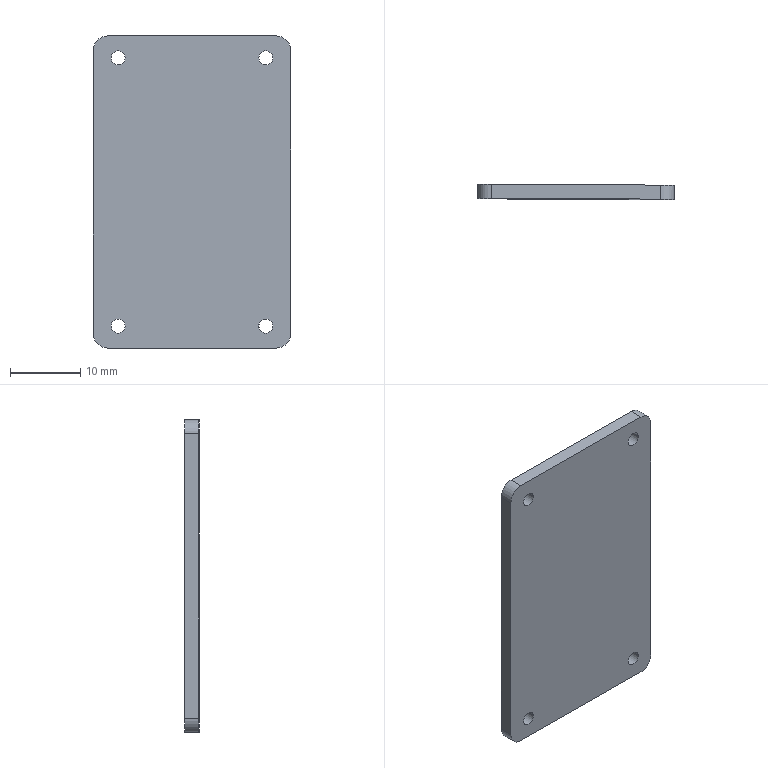Component | SolidWorks | LowerBaffle-1 | 1 solid | 23 faces | box 28.12 x 2.12 x 44.53 mm | volume 2302 mm3 | cylinder 12 | plane 11 | commonest cylinder face diameters 2 x8 4 x4
build123d program:
from build123d import *

# Parameters (mm, degrees)
BOSS_EXTRUDE1_DEPTH = 2
FILLET1_R           = 2
SKETCH2_R           = 1
CUT_EXTRUDE1_DEPTH  = 10
SKETCH3_W           = 14.313
SKETCH3_H           = 23.58
CUT_EXTRUDE2_DEPTH  = 0.5


with BuildPart() as part:
    # Sketch1 → Boss-Extrude1 (new body)
    with BuildSketch(Plane.XY):
        Polygon((102.385, 21.878), (74.276, 21.878), (74.276, -0.3844), (74.276, -22.646), (102.385, -22.646), align=None)
    extrude(amount=BOSS_EXTRUDE1_DEPTH)

    # Fillet1
    fillet1_edges = [part.edges().sort_by_distance(p)[0] for p in [
        (102.385, -22.646, 1),
        (74.276, -22.646, 1),
        (74.276, 21.878, 1),
        (102.385, 21.878, 1),
    ]]
    fillet(fillet1_edges, radius=FILLET1_R)

    # Sketch2 → Cut-Extrude1 (cut)
    with BuildSketch(Plane.XY.offset(2)):
        with Locations((98.864, 18.749)):
            Circle(SKETCH2_R)
        with Locations((77.792, 18.749)):
            Circle(SKETCH2_R)
        with Locations(Location((77.792, -19.518, 0), (0, 0, 180))):
            Circle(SKETCH2_R)
        with Locations(Location((98.864, -19.518, 0), (0, 0, 180))):
            Circle(SKETCH2_R)
    extrude(amount=-CUT_EXTRUDE1_DEPTH, mode=Mode.SUBTRACT)

    # Sketch3 → Cut-Extrude2 (cut)
    with BuildSketch(Plane.XY.offset(2)):
        with Locations((89.245, -0.1111)):
            Rectangle(SKETCH3_W, SKETCH3_H)
    extrude(amount=-CUT_EXTRUDE2_DEPTH, mode=Mode.SUBTRACT)


solid = part.part

# Placed as in the assembly
solid = solid.moved(Location((64.806, 26.824, -0.2506), (-90, 0.2356, 0.008241)))
STEP:
#1=COLOUR_RGB('',0.7922,0.8196,0.9333);
#2=FILL_AREA_STYLE_COLOUR('',#1);
#3=FILL_AREA_STYLE('',(#2));
#4=SURFACE_STYLE_FILL_AREA(#3);
#5=SURFACE_SIDE_STYLE('',(#4));
#6=SURFACE_STYLE_USAGE(.BOTH.,#5);
#7=PRESENTATION_STYLE_ASSIGNMENT((#6));
#8=CARTESIAN_POINT('',(6.483,1.04,0.758));
#9=VERTEX_POINT('',#8);
#10=CARTESIAN_POINT('',(6.404,1.04,0.758));
#11=VERTEX_POINT('',#10);
#12=CARTESIAN_POINT('',(6.444,1.04,0.758));
#13=DIRECTION('',(-0.004111,-1.,0.));
#14=DIRECTION('',(-1.,0.004111,0.0001438));
#15=AXIS2_PLACEMENT_3D('',#12,#13,#14);
#16=CIRCLE('',#15,0.03937);
#17=EDGE_CURVE('',#9,#11,#16,.T.);
#18=ORIENTED_EDGE('',*,*,#17,.T.);
#19=CARTESIAN_POINT('',(6.405,1.119,0.758));
#20=VERTEX_POINT('',#19);
#21=CARTESIAN_POINT('',(6.403,0.7253,0.758));
#22=DIRECTION('',(0.004111,1.,0.));
#23=VECTOR('',#22,39.37);
#24=LINE('',#21,#23);
#25=EDGE_CURVE('',#11,#20,#24,.T.);
#26=ORIENTED_EDGE('',*,*,#25,.T.);
#27=CARTESIAN_POINT('',(6.483,1.119,0.758));
#28=VERTEX_POINT('',#27);
#29=CARTESIAN_POINT('',(6.444,1.119,0.758));
#30=DIRECTION('',(0.004111,1.,0.));
#31=DIRECTION('',(-1.,0.004111,0.0001438));
#32=AXIS2_PLACEMENT_3D('',#29,#30,#31);
#33=CIRCLE('',#32,0.03937);
#34=EDGE_CURVE('',#20,#28,#33,.T.);
#35=ORIENTED_EDGE('',*,*,#34,.T.);
#36=CARTESIAN_POINT('',(6.482,0.7249,0.758));
#37=DIRECTION('',(0.004111,1.,0.));
#38=VECTOR('',#37,39.37);
#39=LINE('',#36,#38);
#40=EDGE_CURVE('',#9,#28,#39,.T.);
#41=ORIENTED_EDGE('',*,*,#40,.F.);
#42=EDGE_LOOP('',(#18,#26,#35,#41));
#43=FACE_OUTER_BOUND('',#42,.T.);
#44=CARTESIAN_POINT('',(6.442,0.7251,0.758));
#45=DIRECTION('',(0.004111,1.,0.));
#46=DIRECTION('',(1.,-0.004111,-0.0001438));
#47=AXIS2_PLACEMENT_3D('',#44,#45,#46);
#48=CYLINDRICAL_SURFACE('',#47,0.03937);
#49=ADVANCED_FACE('',(#43),#48,.F.);
#50=CARTESIAN_POINT('',(5.654,1.043,0.7581));
#51=VERTEX_POINT('',#50);
#52=CARTESIAN_POINT('',(5.575,1.044,0.7581));
#53=VERTEX_POINT('',#52);
#54=CARTESIAN_POINT('',(5.614,1.043,0.7581));
#55=DIRECTION('',(-0.004111,-1.,0.));
#56=DIRECTION('',(-1.,0.004111,0.0001438));
#57=AXIS2_PLACEMENT_3D('',#54,#55,#56);
#58=CIRCLE('',#57,0.03937);
#59=EDGE_CURVE('',#51,#53,#58,.T.);
#60=ORIENTED_EDGE('',*,*,#59,.T.);
#61=CARTESIAN_POINT('',(5.575,1.122,0.7581));
#62=VERTEX_POINT('',#61);
#63=CARTESIAN_POINT('',(5.573,0.7287,0.7581));
#64=DIRECTION('',(0.004111,1.,0.));
#65=VECTOR('',#64,39.37);
#66=LINE('',#63,#65);
#67=EDGE_CURVE('',#53,#62,#66,.T.);
#68=ORIENTED_EDGE('',*,*,#67,.T.);
#69=CARTESIAN_POINT('',(5.654,1.122,0.7581));
#70=VERTEX_POINT('',#69);
#71=CARTESIAN_POINT('',(5.614,1.122,0.7581));
#72=DIRECTION('',(0.004111,1.,0.));
#73=DIRECTION('',(-1.,0.004111,0.0001438));
#74=AXIS2_PLACEMENT_3D('',#71,#72,#73);
#75=CIRCLE('',#74,0.03937);
#76=EDGE_CURVE('',#62,#70,#75,.T.);
#77=ORIENTED_EDGE('',*,*,#76,.T.);
#78=CARTESIAN_POINT('',(5.652,0.7284,0.7581));
#79=DIRECTION('',(0.004111,1.,0.));
#80=VECTOR('',#79,39.37);
#81=LINE('',#78,#80);
#82=EDGE_CURVE('',#51,#70,#81,.T.);
#83=ORIENTED_EDGE('',*,*,#82,.F.);
#84=EDGE_LOOP('',(#60,#68,#77,#83));
#85=FACE_OUTER_BOUND('',#84,.T.);
#86=CARTESIAN_POINT('',(5.613,0.7285,0.7581));
#87=DIRECTION('',(0.004111,1.,0.));
#88=DIRECTION('',(1.,-0.004111,-0.0001438));
#89=AXIS2_PLACEMENT_3D('',#86,#87,#88);
#90=CYLINDRICAL_SURFACE('',#89,0.03937);
#91=ADVANCED_FACE('',(#85),#90,.F.);
#92=CARTESIAN_POINT('',(5.653,1.043,-0.7485));
#93=VERTEX_POINT('',#92);
#94=CARTESIAN_POINT('',(5.575,1.044,-0.7485));
#95=VERTEX_POINT('',#94);
#96=CARTESIAN_POINT('',(5.614,1.043,-0.7485));
#97=DIRECTION('',(-0.004111,-1.,0.));
#98=DIRECTION('',(-1.,0.004111,0.0001438));
#99=AXIS2_PLACEMENT_3D('',#96,#97,#98);
#100=CIRCLE('',#99,0.03937);
#101=EDGE_CURVE('',#93,#95,#100,.T.);
#102=ORIENTED_EDGE('',*,*,#101,.T.);
#103=CARTESIAN_POINT('',(5.575,1.122,-0.7485));
#104=VERTEX_POINT('',#103);
#105=CARTESIAN_POINT('',(5.573,0.7287,-0.7485));
#106=DIRECTION('',(0.004111,1.,0.));
#107=VECTOR('',#106,39.37);
#108=LINE('',#105,#107);
#109=EDGE_CURVE('',#95,#104,#108,.T.);
#110=ORIENTED_EDGE('',*,*,#109,.T.);
#111=CARTESIAN_POINT('',(5.654,1.122,-0.7485));
#112=VERTEX_POINT('',#111);
#113=CARTESIAN_POINT('',(5.614,1.122,-0.7485));
#114=DIRECTION('',(0.004111,1.,0.));
#115=DIRECTION('',(1.,-0.004111,-0.0001438));
#116=AXIS2_PLACEMENT_3D('',#113,#114,#115);
#117=CIRCLE('',#116,0.03937);
#118=EDGE_CURVE('',#104,#112,#117,.T.);
#119=ORIENTED_EDGE('',*,*,#118,.T.);
#120=CARTESIAN_POINT('',(5.652,0.7284,-0.7485));
#121=DIRECTION('',(0.004111,1.,0.));
#122=VECTOR('',#121,39.37);
#123=LINE('',#120,#122);
#124=EDGE_CURVE('',#93,#112,#123,.T.);
#125=ORIENTED_EDGE('',*,*,#124,.F.);
#126=EDGE_LOOP('',(#102,#110,#119,#125));
#127=FACE_OUTER_BOUND('',#126,.T.);
#128=CARTESIAN_POINT('',(5.613,0.7285,-0.7485));
#129=DIRECTION('',(0.004111,1.,0.));
#130=DIRECTION('',(1.,-0.004111,-0.0001438));
#131=AXIS2_PLACEMENT_3D('',#128,#129,#130);
#132=CYLINDRICAL_SURFACE('',#131,0.03937);
#133=ADVANCED_FACE('',(#127),#132,.F.);
#134=CARTESIAN_POINT('',(6.483,1.04,-0.7486));
#135=VERTEX_POINT('',#134);
#136=CARTESIAN_POINT('',(6.404,1.04,-0.7486));
#137=VERTEX_POINT('',#136);
#138=CARTESIAN_POINT('',(6.444,1.04,-0.7486));
#139=DIRECTION('',(-0.004111,-1.,0.));
#140=DIRECTION('',(-1.,0.004111,0.0001438));
#141=AXIS2_PLACEMENT_3D('',#138,#139,#140);
#142=CIRCLE('',#141,0.03937);
#143=EDGE_CURVE('',#135,#137,#142,.T.);
#144=ORIENTED_EDGE('',*,*,#143,.T.);
#145=CARTESIAN_POINT('',(6.405,1.119,-0.7486));
#146=VERTEX_POINT('',#145);
#147=CARTESIAN_POINT('',(6.403,0.7253,-0.7486));
#148=DIRECTION('',(0.004111,1.,0.));
#149=VECTOR('',#148,39.37);
#150=LINE('',#147,#149);
#151=EDGE_CURVE('',#137,#146,#150,.T.);
#152=ORIENTED_EDGE('',*,*,#151,.T.);
#153=CARTESIAN_POINT('',(6.483,1.119,-0.7486));
#154=VERTEX_POINT('',#153);
#155=CARTESIAN_POINT('',(6.444,1.119,-0.7486));
#156=DIRECTION('',(0.004111,1.,0.));
#157=DIRECTION('',(1.,-0.004111,-0.0001438));
#158=AXIS2_PLACEMENT_3D('',#155,#156,#157);
#159=CIRCLE('',#158,0.03937);
#160=EDGE_CURVE('',#146,#154,#159,.T.);
#161=ORIENTED_EDGE('',*,*,#160,.T.);
#162=CARTESIAN_POINT('',(6.482,0.725,-0.7486));
#163=DIRECTION('',(0.004111,1.,0.));
#164=VECTOR('',#163,39.37);
#165=LINE('',#162,#164);
#166=EDGE_CURVE('',#135,#154,#165,.T.);
#167=ORIENTED_EDGE('',*,*,#166,.F.);
#168=EDGE_LOOP('',(#144,#152,#161,#167));
#169=FACE_OUTER_BOUND('',#168,.T.);
#170=CARTESIAN_POINT('',(6.442,0.7251,-0.7486));
#171=DIRECTION('',(0.004111,1.,0.));
#172=DIRECTION('',(1.,-0.004111,-0.0001438));
#173=AXIS2_PLACEMENT_3D('',#170,#171,#172);
#174=CYLINDRICAL_SURFACE('',#173,0.03937);
#175=ADVANCED_FACE('',(#169),#174,.F.);
#176=CARTESIAN_POINT('',(6.583,1.118,0.8024));
#177=VERTEX_POINT('',#176);
#178=CARTESIAN_POINT('',(6.582,1.118,-0.793));
#179=VERTEX_POINT('',#178);
#180=CARTESIAN_POINT('',(6.582,1.118,-0.8718));
#181=DIRECTION('',(-0.0001438,0.00000059,-1.));
#182=VECTOR('',#181,39.37);
#183=LINE('',#180,#182);
#184=EDGE_CURVE('',#177,#179,#183,.T.);
#185=ORIENTED_EDGE('',*,*,#184,.F.);
#186=CARTESIAN_POINT('',(6.582,1.039,0.8024));
#187=VERTEX_POINT('',#186);
#188=CARTESIAN_POINT('',(6.583,1.118,0.8024));
#189=DIRECTION('',(-0.004111,-1.,0.));
#190=VECTOR('',#189,39.37);
#191=LINE('',#188,#190);
#192=EDGE_CURVE('',#177,#187,#191,.T.);
#193=ORIENTED_EDGE('',*,*,#192,.T.);
#194=CARTESIAN_POINT('',(6.582,1.04,-0.793));
#195=VERTEX_POINT('',#194);
#196=CARTESIAN_POINT('',(6.582,1.04,-0.8718));
#197=DIRECTION('',(-0.0001438,0.00000059,-1.));
#198=VECTOR('',#197,39.37);
#199=LINE('',#196,#198);
#200=EDGE_CURVE('',#187,#195,#199,.T.);
#201=ORIENTED_EDGE('',*,*,#200,.T.);
#202=CARTESIAN_POINT('',(6.582,1.118,-0.793));
#203=DIRECTION('',(0.004111,1.,0.));
#204=VECTOR('',#203,39.37);
#205=LINE('',#202,#204);
#206=EDGE_CURVE('',#195,#179,#205,.T.);
#207=ORIENTED_EDGE('',*,*,#206,.T.);
#208=EDGE_LOOP('',(#185,#193,#201,#207));
#209=FACE_OUTER_BOUND('',#208,.T.);
#210=CARTESIAN_POINT('',(6.582,1.118,-0.8718));
#211=DIRECTION('',(-1.,0.004111,0.0001438));
#212=DIRECTION('',(0.004111,1.,0.));
#213=AXIS2_PLACEMENT_3D('',#210,#211,#212);
#214=PLANE('',#213);
#215=ADVANCED_FACE('',(#209),#214,.F.);
#216=CARTESIAN_POINT('',(6.503,1.04,-0.8718));
#217=VERTEX_POINT('',#216);
#218=CARTESIAN_POINT('',(5.554,1.044,-0.8716));
#219=VERTEX_POINT('',#218);
#220=CARTESIAN_POINT('',(6.582,1.04,-0.8718));
#221=DIRECTION('',(-1.,0.004111,0.0001438));
#222=VECTOR('',#221,39.37);
#223=LINE('',#220,#222);
#224=EDGE_CURVE('',#217,#219,#223,.T.);
#225=ORIENTED_EDGE('',*,*,#224,.T.);
#226=CARTESIAN_POINT('',(5.555,1.122,-0.8716));
#227=VERTEX_POINT('',#226);
#228=CARTESIAN_POINT('',(5.555,1.122,-0.8716));
#229=DIRECTION('',(0.004111,1.,0.));
#230=VECTOR('',#229,39.37);
#231=LINE('',#228,#230);
#232=EDGE_CURVE('',#219,#227,#231,.T.);
#233=ORIENTED_EDGE('',*,*,#232,.T.);
#234=CARTESIAN_POINT('',(6.504,1.119,-0.8718));
#235=VERTEX_POINT('',#234);
#236=CARTESIAN_POINT('',(6.582,1.118,-0.8718));
#237=DIRECTION('',(-1.,0.004111,0.0001438));
#238=VECTOR('',#237,39.37);
#239=LINE('',#236,#238);
#240=EDGE_CURVE('',#235,#227,#239,.T.);
#241=ORIENTED_EDGE('',*,*,#240,.F.);
#242=CARTESIAN_POINT('',(6.504,1.119,-0.8718));
#243=DIRECTION('',(-0.004111,-1.,0.));
#244=VECTOR('',#243,39.37);
#245=LINE('',#242,#244);
#246=EDGE_CURVE('',#235,#217,#245,.T.);
#247=ORIENTED_EDGE('',*,*,#246,.T.);
#248=EDGE_LOOP('',(#225,#233,#241,#247));
#249=FACE_OUTER_BOUND('',#248,.T.);
#250=CARTESIAN_POINT('',(6.582,1.118,-0.8718));
#251=DIRECTION('',(0.0001438,-0.00000059,1.));
#252=DIRECTION('',(1.,-0.004111,-0.0001438));
#253=AXIS2_PLACEMENT_3D('',#250,#251,#252);
#254=PLANE('',#253);
#255=ADVANCED_FACE('',(#249),#254,.F.);
#256=CARTESIAN_POINT('',(5.476,1.044,-0.7929));
#257=VERTEX_POINT('',#256);
#258=CARTESIAN_POINT('',(5.476,1.044,0.8026));
#259=VERTEX_POINT('',#258);
#260=CARTESIAN_POINT('',(5.476,1.044,0.004848));
#261=DIRECTION('',(0.0001438,-0.00000059,1.));
#262=VECTOR('',#261,39.37);
#263=LINE('',#260,#262);
#264=EDGE_CURVE('',#257,#259,#263,.T.);
#265=ORIENTED_EDGE('',*,*,#264,.T.);
#266=CARTESIAN_POINT('',(5.476,1.123,0.8026));
#267=VERTEX_POINT('',#266);
#268=CARTESIAN_POINT('',(5.476,1.123,0.8026));
#269=DIRECTION('',(0.004111,1.,0.));
#270=VECTOR('',#269,39.37);
#271=LINE('',#268,#270);
#272=EDGE_CURVE('',#259,#267,#271,.T.);
#273=ORIENTED_EDGE('',*,*,#272,.T.);
#274=CARTESIAN_POINT('',(5.476,1.123,-0.7929));
#275=VERTEX_POINT('',#274);
#276=CARTESIAN_POINT('',(5.476,1.123,-0.8716));
#277=DIRECTION('',(0.0001438,-0.00000059,1.));
#278=VECTOR('',#277,39.37);
#279=LINE('',#276,#278);
#280=EDGE_CURVE('',#275,#267,#279,.T.);
#281=ORIENTED_EDGE('',*,*,#280,.F.);
#282=CARTESIAN_POINT('',(5.476,1.123,-0.7929));
#283=DIRECTION('',(-0.004111,-1.,0.));
#284=VECTOR('',#283,39.37);
#285=LINE('',#282,#284);
#286=EDGE_CURVE('',#275,#257,#285,.T.);
#287=ORIENTED_EDGE('',*,*,#286,.T.);
#288=EDGE_LOOP('',(#265,#273,#281,#287));
#289=FACE_OUTER_BOUND('',#288,.T.);
#290=CARTESIAN_POINT('',(5.476,1.123,0.004848));
#291=DIRECTION('',(1.,-0.004111,-0.0001438));
#292=DIRECTION('',(-0.0001438,0.00000059,-1.));
#293=AXIS2_PLACEMENT_3D('',#290,#291,#292);
#294=PLANE('',#293);
#295=ADVANCED_FACE('',(#289),#294,.F.);
#296=CARTESIAN_POINT('',(5.555,1.122,0.8813));
#297=VERTEX_POINT('',#296);
#298=CARTESIAN_POINT('',(6.504,1.119,0.8812));
#299=VERTEX_POINT('',#298);
#300=CARTESIAN_POINT('',(6.583,1.118,0.8811));
#301=DIRECTION('',(1.,-0.004111,-0.0001438));
#302=VECTOR('',#301,39.37);
#303=LINE('',#300,#302);
#304=EDGE_CURVE('',#297,#299,#303,.T.);
#305=ORIENTED_EDGE('',*,*,#304,.F.);
#306=CARTESIAN_POINT('',(5.554,1.044,0.8813));
#307=VERTEX_POINT('',#306);
#308=CARTESIAN_POINT('',(5.555,1.122,0.8813));
#309=DIRECTION('',(-0.004111,-1.,0.));
#310=VECTOR('',#309,39.37);
#311=LINE('',#308,#310);
#312=EDGE_CURVE('',#297,#307,#311,.T.);
#313=ORIENTED_EDGE('',*,*,#312,.T.);
#314=CARTESIAN_POINT('',(6.504,1.04,0.8812));
#315=VERTEX_POINT('',#314);
#316=CARTESIAN_POINT('',(6.582,1.039,0.8811));
#317=DIRECTION('',(1.,-0.004111,-0.0001438));
#318=VECTOR('',#317,39.37);
#319=LINE('',#316,#318);
#320=EDGE_CURVE('',#307,#315,#319,.T.);
#321=ORIENTED_EDGE('',*,*,#320,.T.);
#322=CARTESIAN_POINT('',(6.504,1.119,0.8812));
#323=DIRECTION('',(0.004111,1.,0.));
#324=VECTOR('',#323,39.37);
#325=LINE('',#322,#324);
#326=EDGE_CURVE('',#315,#299,#325,.T.);
#327=ORIENTED_EDGE('',*,*,#326,.T.);
#328=EDGE_LOOP('',(#305,#313,#321,#327));
#329=FACE_OUTER_BOUND('',#328,.T.);
#330=CARTESIAN_POINT('',(6.583,1.118,0.8811));
#331=DIRECTION('',(-0.0001438,0.00000059,-1.));
#332=DIRECTION('',(-1.,0.004111,0.0001438));
#333=AXIS2_PLACEMENT_3D('',#330,#331,#332);
#334=PLANE('',#333);
#335=ADVANCED_FACE('',(#329),#334,.F.);
#336=CARTESIAN_POINT('',(6.347,1.119,-0.4702));
#337=VERTEX_POINT('',#336);
#338=CARTESIAN_POINT('',(5.783,1.122,-0.4701));
#339=VERTEX_POINT('',#338);
#340=CARTESIAN_POINT('',(6.347,1.119,-0.4702));
#341=DIRECTION('',(-1.,0.004111,0.0001438));
#342=VECTOR('',#341,39.37);
#343=LINE('',#340,#342);
#344=EDGE_CURVE('',#337,#339,#343,.T.);
#345=ORIENTED_EDGE('',*,*,#344,.F.);
#346=CARTESIAN_POINT('',(6.347,1.119,0.4581));
#347=VERTEX_POINT('',#346);
#348=CARTESIAN_POINT('',(6.347,1.119,-0.4702));
#349=DIRECTION('',(-0.0001438,0.00000059,-1.));
#350=VECTOR('',#349,39.37);
#351=LINE('',#348,#350);
#352=EDGE_CURVE('',#347,#337,#351,.T.);
#353=ORIENTED_EDGE('',*,*,#352,.F.);
#354=CARTESIAN_POINT('',(5.784,1.122,0.4582));
#355=VERTEX_POINT('',#354);
#356=CARTESIAN_POINT('',(6.347,1.119,0.4581));
#357=DIRECTION('',(1.,-0.004111,-0.0001438));
#358=VECTOR('',#357,39.37);
#359=LINE('',#356,#358);
#360=EDGE_CURVE('',#355,#347,#359,.T.);
#361=ORIENTED_EDGE('',*,*,#360,.F.);
#362=CARTESIAN_POINT('',(5.783,1.122,-0.4701));
#363=DIRECTION('',(0.0001438,-0.00000059,1.));
#364=VECTOR('',#363,39.37);
#365=LINE('',#362,#364);
#366=EDGE_CURVE('',#339,#355,#365,.T.);
#367=ORIENTED_EDGE('',*,*,#366,.F.);
#368=EDGE_LOOP('',(#345,#353,#361,#367));
#369=FACE_BOUND('',#368,.T.);
#370=CARTESIAN_POINT('',(6.444,1.119,0.758));
#371=DIRECTION('',(0.004111,1.,0.));
#372=DIRECTION('',(-1.,0.004111,0.0001438));
#373=AXIS2_PLACEMENT_3D('',#370,#371,#372);
#374=CIRCLE('',#373,0.03937);
#375=EDGE_CURVE('',#28,#20,#374,.T.);
#376=ORIENTED_EDGE('',*,*,#375,.F.);
#377=ORIENTED_EDGE('',*,*,#34,.F.);
#378=EDGE_LOOP('',(#376,#377));
#379=FACE_BOUND('',#378,.T.);
#380=CARTESIAN_POINT('',(5.614,1.122,0.7581));
#381=DIRECTION('',(0.004111,1.,0.));
#382=DIRECTION('',(-1.,0.004111,0.0001438));
#383=AXIS2_PLACEMENT_3D('',#380,#381,#382);
#384=CIRCLE('',#383,0.03937);
#385=EDGE_CURVE('',#70,#62,#384,.T.);
#386=ORIENTED_EDGE('',*,*,#385,.F.);
#387=ORIENTED_EDGE('',*,*,#76,.F.);
#388=EDGE_LOOP('',(#386,#387));
#389=FACE_BOUND('',#388,.T.);
#390=CARTESIAN_POINT('',(5.614,1.122,-0.7485));
#391=DIRECTION('',(0.004111,1.,0.));
#392=DIRECTION('',(1.,-0.004111,-0.0001438));
#393=AXIS2_PLACEMENT_3D('',#390,#391,#392);
#394=CIRCLE('',#393,0.03937);
#395=EDGE_CURVE('',#112,#104,#394,.T.);
#396=ORIENTED_EDGE('',*,*,#395,.F.);
#397=ORIENTED_EDGE('',*,*,#118,.F.);
#398=EDGE_LOOP('',(#396,#397));
#399=FACE_BOUND('',#398,.T.);
#400=CARTESIAN_POINT('',(6.444,1.119,-0.7486));
#401=DIRECTION('',(0.004111,1.,0.));
#402=DIRECTION('',(1.,-0.004111,-0.0001438));
#403=AXIS2_PLACEMENT_3D('',#400,#401,#402);
#404=CIRCLE('',#403,0.03937);
#405=EDGE_CURVE('',#154,#146,#404,.T.);
#406=ORIENTED_EDGE('',*,*,#405,.F.);
#407=ORIENTED_EDGE('',*,*,#160,.F.);
#408=EDGE_LOOP('',(#406,#407));
#409=FACE_BOUND('',#408,.T.);
#410=ORIENTED_EDGE('',*,*,#280,.T.);
#411=CARTESIAN_POINT('',(5.555,1.122,0.8026));
#412=DIRECTION('',(0.004111,1.,0.));
#413=DIRECTION('',(-1.,0.004111,0.0001438));
#414=AXIS2_PLACEMENT_3D('',#411,#412,#413);
#415=CIRCLE('',#414,0.07874);
#416=EDGE_CURVE('',#267,#297,#415,.T.);
#417=ORIENTED_EDGE('',*,*,#416,.T.);
#418=ORIENTED_EDGE('',*,*,#304,.T.);
#419=CARTESIAN_POINT('',(6.504,1.119,0.8024));
#420=DIRECTION('',(0.004111,1.,0.));
#421=DIRECTION('',(-1.,0.004111,0.0001438));
#422=AXIS2_PLACEMENT_3D('',#419,#420,#421);
#423=CIRCLE('',#422,0.07874);
#424=EDGE_CURVE('',#299,#177,#423,.T.);
#425=ORIENTED_EDGE('',*,*,#424,.T.);
#426=ORIENTED_EDGE('',*,*,#184,.T.);
#427=CARTESIAN_POINT('',(6.504,1.119,-0.793));
#428=DIRECTION('',(0.004111,1.,0.));
#429=DIRECTION('',(-1.,0.004111,0.0001438));
#430=AXIS2_PLACEMENT_3D('',#427,#428,#429);
#431=CIRCLE('',#430,0.07874);
#432=EDGE_CURVE('',#179,#235,#431,.T.);
#433=ORIENTED_EDGE('',*,*,#432,.T.);
#434=ORIENTED_EDGE('',*,*,#240,.T.);
#435=CARTESIAN_POINT('',(5.555,1.122,-0.7929));
#436=DIRECTION('',(0.004111,1.,0.));
#437=DIRECTION('',(-1.,0.004111,0.0001438));
#438=AXIS2_PLACEMENT_3D('',#435,#436,#437);
#439=CIRCLE('',#438,0.07874);
#440=EDGE_CURVE('',#227,#275,#439,.T.);
#441=ORIENTED_EDGE('',*,*,#440,.T.);
#442=EDGE_LOOP('',(#410,#417,#418,#425,#426,#433,#434,#441));
#443=FACE_OUTER_BOUND('',#442,.T.);
#444=CARTESIAN_POINT('',(2.552,1.135,-0.009864));
#445=DIRECTION('',(-0.004111,-1.,0.));
#446=DIRECTION('',(-1.,0.004111,0.0001438));
#447=AXIS2_PLACEMENT_3D('',#444,#445,#446);
#448=PLANE('',#447);
#449=ADVANCED_FACE('',(#369,#379,#389,#399,#409,#443),#448,.F.);
#450=ORIENTED_EDGE('',*,*,#17,.F.);
#451=CARTESIAN_POINT('',(6.444,1.04,0.758));
#452=DIRECTION('',(-0.004111,-1.,0.));
#453=DIRECTION('',(-1.,0.004111,0.0001438));
#454=AXIS2_PLACEMENT_3D('',#451,#452,#453);
#455=CIRCLE('',#454,0.03937);
#456=EDGE_CURVE('',#11,#9,#455,.T.);
#457=ORIENTED_EDGE('',*,*,#456,.F.);
#458=EDGE_LOOP('',(#450,#457));
#459=FACE_BOUND('',#458,.T.);
#460=ORIENTED_EDGE('',*,*,#59,.F.);
#461=CARTESIAN_POINT('',(5.614,1.043,0.7581));
#462=DIRECTION('',(-0.004111,-1.,0.));
#463=DIRECTION('',(-1.,0.004111,0.0001438));
#464=AXIS2_PLACEMENT_3D('',#461,#462,#463);
#465=CIRCLE('',#464,0.03937);
#466=EDGE_CURVE('',#53,#51,#465,.T.);
#467=ORIENTED_EDGE('',*,*,#466,.F.);
#468=EDGE_LOOP('',(#460,#467));
#469=FACE_BOUND('',#468,.T.);
#470=ORIENTED_EDGE('',*,*,#101,.F.);
#471=CARTESIAN_POINT('',(5.614,1.043,-0.7485));
#472=DIRECTION('',(-0.004111,-1.,0.));
#473=DIRECTION('',(-1.,0.004111,0.0001438));
#474=AXIS2_PLACEMENT_3D('',#471,#472,#473);
#475=CIRCLE('',#474,0.03937);
#476=EDGE_CURVE('',#95,#93,#475,.T.);
#477=ORIENTED_EDGE('',*,*,#476,.F.);
#478=EDGE_LOOP('',(#470,#477));
#479=FACE_BOUND('',#478,.T.);
#480=ORIENTED_EDGE('',*,*,#143,.F.);
#481=CARTESIAN_POINT('',(6.444,1.04,-0.7486));
#482=DIRECTION('',(-0.004111,-1.,0.));
#483=DIRECTION('',(-1.,0.004111,0.0001438));
#484=AXIS2_PLACEMENT_3D('',#481,#482,#483);
#485=CIRCLE('',#484,0.03937);
#486=EDGE_CURVE('',#137,#135,#485,.T.);
#487=ORIENTED_EDGE('',*,*,#486,.F.);
#488=EDGE_LOOP('',(#480,#487));
#489=FACE_BOUND('',#488,.T.);
#490=ORIENTED_EDGE('',*,*,#320,.F.);
#491=CARTESIAN_POINT('',(5.554,1.044,0.8026));
#492=DIRECTION('',(-0.004111,-1.,0.));
#493=DIRECTION('',(-1.,0.004111,0.0001438));
#494=AXIS2_PLACEMENT_3D('',#491,#492,#493);
#495=CIRCLE('',#494,0.07874);
#496=EDGE_CURVE('',#307,#259,#495,.T.);
#497=ORIENTED_EDGE('',*,*,#496,.T.);
#498=ORIENTED_EDGE('',*,*,#264,.F.);
#499=CARTESIAN_POINT('',(5.554,1.044,-0.7929));
#500=DIRECTION('',(-0.004111,-1.,0.));
#501=DIRECTION('',(-1.,0.004111,0.0001438));
#502=AXIS2_PLACEMENT_3D('',#499,#500,#501);
#503=CIRCLE('',#502,0.07874);
#504=EDGE_CURVE('',#257,#219,#503,.T.);
#505=ORIENTED_EDGE('',*,*,#504,.T.);
#506=ORIENTED_EDGE('',*,*,#224,.F.);
#507=CARTESIAN_POINT('',(6.503,1.04,-0.793));
#508=DIRECTION('',(-0.004111,-1.,0.));
#509=DIRECTION('',(-1.,0.004111,0.0001438));
#510=AXIS2_PLACEMENT_3D('',#507,#508,#509);
#511=CIRCLE('',#510,0.07874);
#512=EDGE_CURVE('',#217,#195,#511,.T.);
#513=ORIENTED_EDGE('',*,*,#512,.T.);
#514=ORIENTED_EDGE('',*,*,#200,.F.);
#515=CARTESIAN_POINT('',(6.504,1.04,0.8024));
#516=DIRECTION('',(-0.004111,-1.,0.));
#517=DIRECTION('',(-1.,0.004111,0.0001438));
#518=AXIS2_PLACEMENT_3D('',#515,#516,#517);
#519=CIRCLE('',#518,0.07874);
#520=EDGE_CURVE('',#187,#315,#519,.T.);
#521=ORIENTED_EDGE('',*,*,#520,.T.);
#522=EDGE_LOOP('',(#490,#497,#498,#505,#506,#513,#514,#521));
#523=FACE_OUTER_BOUND('',#522,.T.);
#524=CARTESIAN_POINT('',(2.551,1.056,-0.009864));
#525=DIRECTION('',(-0.004111,-1.,0.));
#526=DIRECTION('',(-1.,0.004111,0.0001438));
#527=AXIS2_PLACEMENT_3D('',#524,#525,#526);
#528=PLANE('',#527);
#529=ADVANCED_FACE('',(#459,#469,#479,#489,#523),#528,.T.);
#530=ORIENTED_EDGE('',*,*,#416,.F.);
#531=ORIENTED_EDGE('',*,*,#272,.F.);
#532=ORIENTED_EDGE('',*,*,#496,.F.);
#533=ORIENTED_EDGE('',*,*,#312,.F.);
#534=EDGE_LOOP('',(#530,#531,#532,#533));
#535=FACE_OUTER_BOUND('',#534,.T.);
#536=CARTESIAN_POINT('',(5.555,1.122,0.8026));
#537=DIRECTION('',(-0.004111,-1.,0.));
#538=DIRECTION('',(-1.,0.004111,0.0001438));
#539=AXIS2_PLACEMENT_3D('',#536,#537,#538);
#540=CYLINDRICAL_SURFACE('',#539,0.07874);
#541=ADVANCED_FACE('',(#535),#540,.T.);
#542=ORIENTED_EDGE('',*,*,#440,.F.);
#543=ORIENTED_EDGE('',*,*,#232,.F.);
#544=ORIENTED_EDGE('',*,*,#504,.F.);
#545=ORIENTED_EDGE('',*,*,#286,.F.);
#546=EDGE_LOOP('',(#542,#543,#544,#545));
#547=FACE_OUTER_BOUND('',#546,.T.);
#548=CARTESIAN_POINT('',(5.555,1.122,-0.7929));
#549=DIRECTION('',(-0.004111,-1.,0.));
#550=DIRECTION('',(-1.,0.004111,0.0001438));
#551=AXIS2_PLACEMENT_3D('',#548,#549,#550);
#552=CYLINDRICAL_SURFACE('',#551,0.07874);
#553=ADVANCED_FACE('',(#547),#552,.T.);
#554=ORIENTED_EDGE('',*,*,#424,.F.);
#555=ORIENTED_EDGE('',*,*,#326,.F.);
#556=ORIENTED_EDGE('',*,*,#520,.F.);
#557=ORIENTED_EDGE('',*,*,#192,.F.);
#558=EDGE_LOOP('',(#554,#555,#556,#557));
#559=FACE_OUTER_BOUND('',#558,.T.);
#560=CARTESIAN_POINT('',(6.504,1.119,0.8024));
#561=DIRECTION('',(-0.004111,-1.,0.));
#562=DIRECTION('',(-1.,0.004111,0.0001438));
#563=AXIS2_PLACEMENT_3D('',#560,#561,#562);
#564=CYLINDRICAL_SURFACE('',#563,0.07874);
#565=ADVANCED_FACE('',(#559),#564,.T.);
#566=ORIENTED_EDGE('',*,*,#432,.F.);
#567=ORIENTED_EDGE('',*,*,#206,.F.);
#568=ORIENTED_EDGE('',*,*,#512,.F.);
#569=ORIENTED_EDGE('',*,*,#246,.F.);
#570=EDGE_LOOP('',(#566,#567,#568,#569));
#571=FACE_OUTER_BOUND('',#570,.T.);
#572=CARTESIAN_POINT('',(6.504,1.119,-0.793));
#573=DIRECTION('',(-0.004111,-1.,0.));
#574=DIRECTION('',(-1.,0.004111,0.0001438));
#575=AXIS2_PLACEMENT_3D('',#572,#573,#574);
#576=CYLINDRICAL_SURFACE('',#575,0.07874);
#577=ADVANCED_FACE('',(#571),#576,.T.);
#578=ORIENTED_EDGE('',*,*,#151,.F.);
#579=ORIENTED_EDGE('',*,*,#486,.T.);
#580=ORIENTED_EDGE('',*,*,#166,.T.);
#581=ORIENTED_EDGE('',*,*,#405,.T.);
#582=EDGE_LOOP('',(#578,#579,#580,#581));
#583=FACE_OUTER_BOUND('',#582,.T.);
#584=CARTESIAN_POINT('',(6.442,0.7251,-0.7486));
#585=DIRECTION('',(0.004111,1.,0.));
#586=DIRECTION('',(1.,-0.004111,-0.0001438));
#587=AXIS2_PLACEMENT_3D('',#584,#585,#586);
#588=CYLINDRICAL_SURFACE('',#587,0.03937);
#589=ADVANCED_FACE('',(#583),#588,.F.);
#590=ORIENTED_EDGE('',*,*,#109,.F.);
#591=ORIENTED_EDGE('',*,*,#476,.T.);
#592=ORIENTED_EDGE('',*,*,#124,.T.);
#593=ORIENTED_EDGE('',*,*,#395,.T.);
#594=EDGE_LOOP('',(#590,#591,#592,#593));
#595=FACE_OUTER_BOUND('',#594,.T.);
#596=CARTESIAN_POINT('',(5.613,0.7285,-0.7485));
#597=DIRECTION('',(0.004111,1.,0.));
#598=DIRECTION('',(1.,-0.004111,-0.0001438));
#599=AXIS2_PLACEMENT_3D('',#596,#597,#598);
#600=CYLINDRICAL_SURFACE('',#599,0.03937);
#601=ADVANCED_FACE('',(#595),#600,.F.);
#602=ORIENTED_EDGE('',*,*,#67,.F.);
#603=ORIENTED_EDGE('',*,*,#466,.T.);
#604=ORIENTED_EDGE('',*,*,#82,.T.);
#605=ORIENTED_EDGE('',*,*,#385,.T.);
#606=EDGE_LOOP('',(#602,#603,#604,#605));
#607=FACE_OUTER_BOUND('',#606,.T.);
#608=CARTESIAN_POINT('',(5.613,0.7285,0.7581));
#609=DIRECTION('',(0.004111,1.,0.));
#610=DIRECTION('',(1.,-0.004111,-0.0001438));
#611=AXIS2_PLACEMENT_3D('',#608,#609,#610);
#612=CYLINDRICAL_SURFACE('',#611,0.03937);
#613=ADVANCED_FACE('',(#607),#612,.F.);
#614=ORIENTED_EDGE('',*,*,#25,.F.);
#615=ORIENTED_EDGE('',*,*,#456,.T.);
#616=ORIENTED_EDGE('',*,*,#40,.T.);
#617=ORIENTED_EDGE('',*,*,#375,.T.);
#618=EDGE_LOOP('',(#614,#615,#616,#617));
#619=FACE_OUTER_BOUND('',#618,.T.);
#620=CARTESIAN_POINT('',(6.442,0.7251,0.758));
#621=DIRECTION('',(0.004111,1.,0.));
#622=DIRECTION('',(1.,-0.004111,-0.0001438));
#623=AXIS2_PLACEMENT_3D('',#620,#621,#622);
#624=CYLINDRICAL_SURFACE('',#623,0.03937);
#625=ADVANCED_FACE('',(#619),#624,.F.);
#626=ORIENTED_EDGE('',*,*,#352,.T.);
#627=CARTESIAN_POINT('',(6.347,1.1,-0.4702));
#628=VERTEX_POINT('',#627);
#629=CARTESIAN_POINT('',(6.347,1.1,-0.4702));
#630=DIRECTION('',(0.004111,1.,0.));
#631=VECTOR('',#630,39.37);
#632=LINE('',#629,#631);
#633=EDGE_CURVE('',#628,#337,#632,.T.);
#634=ORIENTED_EDGE('',*,*,#633,.F.);
#635=CARTESIAN_POINT('',(6.347,1.1,0.4581));
#636=VERTEX_POINT('',#635);
#637=CARTESIAN_POINT('',(6.347,1.1,-0.4702));
#638=DIRECTION('',(-0.0001438,0.00000059,-1.));
#639=VECTOR('',#638,39.37);
#640=LINE('',#637,#639);
#641=EDGE_CURVE('',#636,#628,#640,.T.);
#642=ORIENTED_EDGE('',*,*,#641,.F.);
#643=CARTESIAN_POINT('',(6.347,1.1,0.4581));
#644=DIRECTION('',(0.004111,1.,0.));
#645=VECTOR('',#644,39.37);
#646=LINE('',#643,#645);
#647=EDGE_CURVE('',#636,#347,#646,.T.);
#648=ORIENTED_EDGE('',*,*,#647,.T.);
#649=EDGE_LOOP('',(#626,#634,#642,#648));
#650=FACE_OUTER_BOUND('',#649,.T.);
#651=CARTESIAN_POINT('',(6.347,1.1,-0.4702));
#652=DIRECTION('',(1.,-0.004111,-0.0001438));
#653=DIRECTION('',(-0.004111,-1.,0.));
#654=AXIS2_PLACEMENT_3D('',#651,#652,#653);
#655=PLANE('',#654);
#656=ADVANCED_FACE('',(#650),#655,.F.);
#657=ORIENTED_EDGE('',*,*,#360,.T.);
#658=ORIENTED_EDGE('',*,*,#647,.F.);
#659=CARTESIAN_POINT('',(5.784,1.102,0.4582));
#660=VERTEX_POINT('',#659);
#661=CARTESIAN_POINT('',(6.347,1.1,0.4581));
#662=DIRECTION('',(1.,-0.004111,-0.0001438));
#663=VECTOR('',#662,39.37);
#664=LINE('',#661,#663);
#665=EDGE_CURVE('',#660,#636,#664,.T.);
#666=ORIENTED_EDGE('',*,*,#665,.F.);
#667=CARTESIAN_POINT('',(5.784,1.102,0.4582));
#668=DIRECTION('',(0.004111,1.,0.));
#669=VECTOR('',#668,39.37);
#670=LINE('',#667,#669);
#671=EDGE_CURVE('',#660,#355,#670,.T.);
#672=ORIENTED_EDGE('',*,*,#671,.T.);
#673=EDGE_LOOP('',(#657,#658,#666,#672));
#674=FACE_OUTER_BOUND('',#673,.T.);
#675=CARTESIAN_POINT('',(6.347,1.1,0.4581));
#676=DIRECTION('',(0.0001438,-0.00000059,1.));
#677=DIRECTION('',(-0.004111,-1.,0.));
#678=AXIS2_PLACEMENT_3D('',#675,#676,#677);
#679=PLANE('',#678);
#680=ADVANCED_FACE('',(#674),#679,.F.);
#681=ORIENTED_EDGE('',*,*,#366,.T.);
#682=ORIENTED_EDGE('',*,*,#671,.F.);
#683=CARTESIAN_POINT('',(5.783,1.102,-0.4701));
#684=VERTEX_POINT('',#683);
#685=CARTESIAN_POINT('',(5.783,1.102,-0.4701));
#686=DIRECTION('',(0.0001438,-0.00000059,1.));
#687=VECTOR('',#686,39.37);
#688=LINE('',#685,#687);
#689=EDGE_CURVE('',#684,#660,#688,.T.);
#690=ORIENTED_EDGE('',*,*,#689,.F.);
#691=CARTESIAN_POINT('',(5.783,1.102,-0.4701));
#692=DIRECTION('',(0.004111,1.,0.));
#693=VECTOR('',#692,39.37);
#694=LINE('',#691,#693);
#695=EDGE_CURVE('',#684,#339,#694,.T.);
#696=ORIENTED_EDGE('',*,*,#695,.T.);
#697=EDGE_LOOP('',(#681,#682,#690,#696));
#698=FACE_OUTER_BOUND('',#697,.T.);
#699=CARTESIAN_POINT('',(5.783,1.102,-0.4701));
#700=DIRECTION('',(-1.,0.004111,0.0001438));
#701=DIRECTION('',(0.004111,1.,0.));
#702=AXIS2_PLACEMENT_3D('',#699,#700,#701);
#703=PLANE('',#702);
#704=ADVANCED_FACE('',(#698),#703,.F.);
#705=ORIENTED_EDGE('',*,*,#344,.T.);
#706=ORIENTED_EDGE('',*,*,#695,.F.);
#707=CARTESIAN_POINT('',(6.347,1.1,-0.4702));
#708=DIRECTION('',(-1.,0.004111,0.0001438));
#709=VECTOR('',#708,39.37);
#710=LINE('',#707,#709);
#711=EDGE_CURVE('',#628,#684,#710,.T.);
#712=ORIENTED_EDGE('',*,*,#711,.F.);
#713=ORIENTED_EDGE('',*,*,#633,.T.);
#714=EDGE_LOOP('',(#705,#706,#712,#713));
#715=FACE_OUTER_BOUND('',#714,.T.);
#716=CARTESIAN_POINT('',(6.347,1.1,-0.4702));
#717=DIRECTION('',(-0.0001438,0.00000059,-1.));
#718=DIRECTION('',(0.004111,1.,0.));
#719=AXIS2_PLACEMENT_3D('',#716,#717,#718);
#720=PLANE('',#719);
#721=ADVANCED_FACE('',(#715),#720,.F.);
#722=ORIENTED_EDGE('',*,*,#641,.T.);
#723=ORIENTED_EDGE('',*,*,#711,.T.);
#724=ORIENTED_EDGE('',*,*,#689,.T.);
#725=ORIENTED_EDGE('',*,*,#665,.T.);
#726=EDGE_LOOP('',(#722,#723,#724,#725));
#727=FACE_OUTER_BOUND('',#726,.T.);
#728=CARTESIAN_POINT('',(2.552,1.115,-0.009864));
#729=DIRECTION('',(-0.004111,-1.,0.));
#730=DIRECTION('',(-1.,0.004111,0.0001438));
#731=AXIS2_PLACEMENT_3D('',#728,#729,#730);
#732=PLANE('',#731);
#733=ADVANCED_FACE('',(#727),#732,.F.);
#734=CLOSED_SHELL('',(#49,#91,#133,#175,#215,#255,#295,#335,#449,#529,#541,#553,#565,#577,#589,#601,#613,#625,#656,#680,#704,#721,#733));
#735=MANIFOLD_SOLID_BREP('',#734);
#736=STYLED_ITEM('',(#7),#735);
#737=PRESENTATION_LAYER_ASSIGNMENT('','',(#736));
#738=(LENGTH_UNIT()NAMED_UNIT(*)SI_UNIT($,.METRE.));
#739=LENGTH_MEASURE_WITH_UNIT(LENGTH_MEASURE(0.0254),#738);
#740=DIMENSIONAL_EXPONENTS(1.,0.,0.,0.,0.,0.,0.);
#741=(CONVERSION_BASED_UNIT('',#739)LENGTH_UNIT()NAMED_UNIT(#740));
#742=UNCERTAINTY_MEASURE_WITH_UNIT(LENGTH_MEASURE(0.00001),#741,'','');
#743=(NAMED_UNIT(*)PLANE_ANGLE_UNIT()SI_UNIT($,.RADIAN.));
#744=(NAMED_UNIT(*)SI_UNIT($,.STERADIAN.)SOLID_ANGLE_UNIT());
#745=(GEOMETRIC_REPRESENTATION_CONTEXT(3)GLOBAL_UNCERTAINTY_ASSIGNED_CONTEXT((#742))GLOBAL_UNIT_ASSIGNED_CONTEXT((#741,#743,#744))REPRESENTATION_CONTEXT('',''));
#746=MECHANICAL_DESIGN_GEOMETRIC_PRESENTATION_REPRESENTATION('',(#736),#745);
#747=CARTESIAN_POINT('',(0.,0.,0.));
#748=DIRECTION('',(0.,0.,1.));
#749=DIRECTION('',(1.,0.,0.));
#750=AXIS2_PLACEMENT_3D('',#747,#748,#749);
#751=(LENGTH_UNIT()NAMED_UNIT(*)SI_UNIT($,.METRE.));
#752=LENGTH_MEASURE_WITH_UNIT(LENGTH_MEASURE(0.0254),#751);
#753=DIMENSIONAL_EXPONENTS(1.,0.,0.,0.,0.,0.,0.);
#754=(CONVERSION_BASED_UNIT('',#752)LENGTH_UNIT()NAMED_UNIT(#753));
#755=UNCERTAINTY_MEASURE_WITH_UNIT(LENGTH_MEASURE(0.00001),#754,'','');
#756=(NAMED_UNIT(*)PLANE_ANGLE_UNIT()SI_UNIT($,.RADIAN.));
#757=(NAMED_UNIT(*)SI_UNIT($,.STERADIAN.)SOLID_ANGLE_UNIT());
#758=(GEOMETRIC_REPRESENTATION_CONTEXT(3)GLOBAL_UNCERTAINTY_ASSIGNED_CONTEXT((#755))GLOBAL_UNIT_ASSIGNED_CONTEXT((#754,#756,#757))REPRESENTATION_CONTEXT('',''));
#759=ADVANCED_BREP_SHAPE_REPRESENTATION('',(#735,#750),#758);